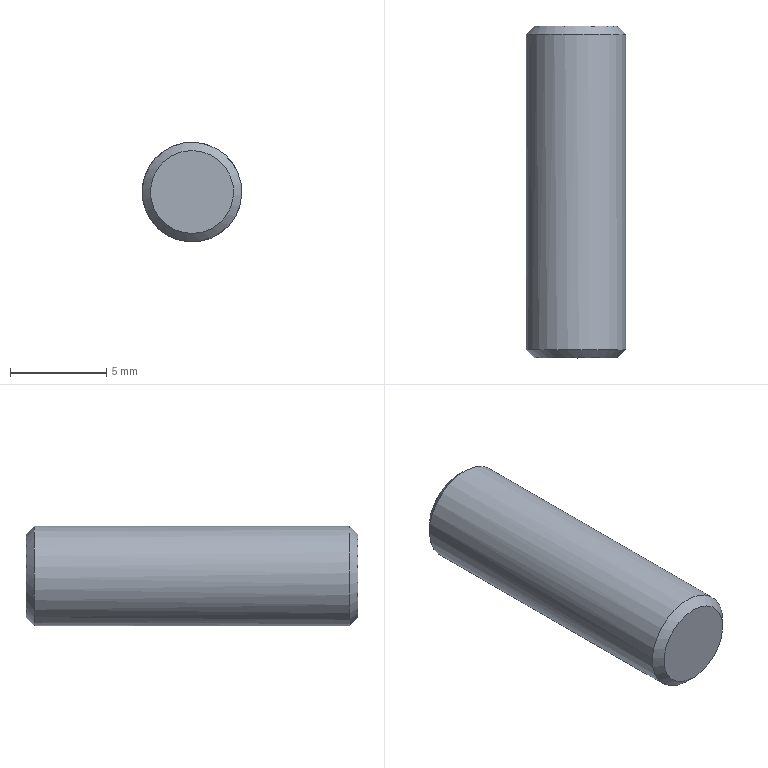Component | NX | 6_LOCATING_PIN | 1 solid | 5 faces | box 5.16 x 17.2 x 5.16 mm | volume 357 mm3 | plane 2 | cone 2 | cylinder 1 | commonest cylinder face diameters 5.16 x1
STEP:
#1=CARTESIAN_POINT('',(0.,0.,0.));
#2=DIRECTION('',(0.,0.,1.));
#3=DIRECTION('',(1.,0.,0.));
#4=AXIS2_PLACEMENT_3D('',#1,#2,#3);
#5=CARTESIAN_POINT('',(-93.38,-477.073,-34.452));
#6=VERTEX_POINT('',#5);
#7=CARTESIAN_POINT('',(-95.366,-477.073,-35.275));
#8=DIRECTION('',(0.,1.,0.));
#9=DIRECTION('',(0.9237,0.,0.383));
#10=AXIS2_PLACEMENT_3D('',#7,#8,#9);
#11=CIRCLE('',#10,2.15);
#12=CARTESIAN_POINT('',(-95.366,-477.073,-35.275));
#13=DIRECTION('',(0.,1.,0.));
#14=DIRECTION('',(0.9237,0.,0.383));
#15=AXIS2_PLACEMENT_3D('',#12,#13,#14);
#16=PLANE('',#15);
#17=CARTESIAN_POINT('',(0.,0.));
#18=DIRECTION('',(1.,-0.));
#19=AXIS2_PLACEMENT_2D('',#17,#18);
#20=CIRCLE('',#19,2.15);
#21=(GEOMETRIC_REPRESENTATION_CONTEXT(2)PARAMETRIC_REPRESENTATION_CONTEXT()REPRESENTATION_CONTEXT('',''));
#22=DEFINITIONAL_REPRESENTATION('',(#20),#21);
#23=PCURVE('',#16,#22);
#24=CARTESIAN_POINT('',(-95.366,-477.503,-35.275));
#25=DIRECTION('',(0.,-1.,0.));
#26=DIRECTION('',(-0.9237,0.,-0.383));
#27=AXIS2_PLACEMENT_3D('',#24,#25,#26);
#28=CONICAL_SURFACE('',#27,2.58,0.7854);
#29=CARTESIAN_POINT('',(9.425,-0.43));
#30=DIRECTION('',(-1.,0.));
#31=VECTOR('',#30,1.);
#32=LINE('',#29,#31);
#33=(GEOMETRIC_REPRESENTATION_CONTEXT(2)PARAMETRIC_REPRESENTATION_CONTEXT()REPRESENTATION_CONTEXT('',''));
#34=DEFINITIONAL_REPRESENTATION('',(#32),#33);
#35=PCURVE('',#28,#34);
#36=SURFACE_CURVE('',#11,(#23,#35),.PCURVE_S1.);
#37=EDGE_CURVE('',#6,#6,#36,.T.);
#38=ORIENTED_EDGE('',*,*,#37,.T.);
#39=EDGE_LOOP('',(#38));
#40=FACE_BOUND('',#39,.T.);
#41=ADVANCED_FACE('',(#40),#16,.T.);
#42=CARTESIAN_POINT('',(-97.352,-494.273,-36.099));
#43=VERTEX_POINT('',#42);
#44=CARTESIAN_POINT('',(-95.366,-494.273,-35.275));
#45=DIRECTION('',(0.,-1.,0.));
#46=DIRECTION('',(-0.9237,0.,-0.383));
#47=AXIS2_PLACEMENT_3D('',#44,#45,#46);
#48=CIRCLE('',#47,2.15);
#49=CARTESIAN_POINT('',(-95.366,-494.273,-35.275));
#50=DIRECTION('',(0.,-1.,0.));
#51=DIRECTION('',(-0.9237,0.,-0.383));
#52=AXIS2_PLACEMENT_3D('',#49,#50,#51);
#53=PLANE('',#52);
#54=CARTESIAN_POINT('',(0.,0.));
#55=DIRECTION('',(1.,0.));
#56=AXIS2_PLACEMENT_2D('',#54,#55);
#57=CIRCLE('',#56,2.15);
#58=(GEOMETRIC_REPRESENTATION_CONTEXT(2)PARAMETRIC_REPRESENTATION_CONTEXT()REPRESENTATION_CONTEXT('',''));
#59=DEFINITIONAL_REPRESENTATION('',(#57),#58);
#60=PCURVE('',#53,#59);
#61=CARTESIAN_POINT('',(-95.366,-493.843,-35.275));
#62=DIRECTION('',(0.,1.,0.));
#63=DIRECTION('',(0.9237,0.,0.383));
#64=AXIS2_PLACEMENT_3D('',#61,#62,#63);
#65=CONICAL_SURFACE('',#64,2.58,0.7854);
#66=CARTESIAN_POINT('',(9.425,-0.43));
#67=DIRECTION('',(-1.,0.));
#68=VECTOR('',#67,1.);
#69=LINE('',#66,#68);
#70=(GEOMETRIC_REPRESENTATION_CONTEXT(2)PARAMETRIC_REPRESENTATION_CONTEXT()REPRESENTATION_CONTEXT('',''));
#71=DEFINITIONAL_REPRESENTATION('',(#69),#70);
#72=PCURVE('',#65,#71);
#73=SURFACE_CURVE('',#48,(#60,#72),.PCURVE_S1.);
#74=EDGE_CURVE('',#43,#43,#73,.T.);
#75=ORIENTED_EDGE('',*,*,#74,.T.);
#76=EDGE_LOOP('',(#75));
#77=FACE_BOUND('',#76,.T.);
#78=ADVANCED_FACE('',(#77),#53,.T.);
#79=CARTESIAN_POINT('',(-97.749,-493.843,-36.264));
#80=VERTEX_POINT('',#79);
#81=CARTESIAN_POINT('',(-92.982,-493.843,-34.287));
#82=VERTEX_POINT('',#81);
#83=CARTESIAN_POINT('',(-95.366,-493.843,-35.275));
#84=DIRECTION('',(0.,1.,0.));
#85=DIRECTION('',(-0.9237,0.,-0.383));
#86=AXIS2_PLACEMENT_3D('',#83,#84,#85);
#87=CIRCLE('',#86,2.58);
#88=CARTESIAN_POINT('',(-95.366,-494.273,-35.275));
#89=DIRECTION('',(0.,1.,0.));
#90=DIRECTION('',(0.9237,0.,0.383));
#91=AXIS2_PLACEMENT_3D('',#88,#89,#90);
#92=CYLINDRICAL_SURFACE('',#91,2.58);
#93=CARTESIAN_POINT('',(3.142,0.43));
#94=DIRECTION('',(1.,0.));
#95=VECTOR('',#94,1.);
#96=LINE('',#93,#95);
#97=(GEOMETRIC_REPRESENTATION_CONTEXT(2)PARAMETRIC_REPRESENTATION_CONTEXT()REPRESENTATION_CONTEXT('',''));
#98=DEFINITIONAL_REPRESENTATION('',(#96),#97);
#99=PCURVE('',#92,#98);
#100=CARTESIAN_POINT('',(3.142,0.));
#101=DIRECTION('',(1.,0.));
#102=VECTOR('',#101,1.);
#103=LINE('',#100,#102);
#104=(GEOMETRIC_REPRESENTATION_CONTEXT(2)PARAMETRIC_REPRESENTATION_CONTEXT()REPRESENTATION_CONTEXT('',''));
#105=DEFINITIONAL_REPRESENTATION('',(#103),#104);
#106=PCURVE('',#65,#105);
#107=SURFACE_CURVE('',#87,(#99,#106),.PCURVE_S1.);
#108=EDGE_CURVE('',#80,#82,#107,.T.);
#109=ORIENTED_EDGE('',*,*,#108,.T.);
#110=CARTESIAN_POINT('',(-92.982,-477.503,-34.287));
#111=VERTEX_POINT('',#110);
#112=CARTESIAN_POINT('',(-92.982,-493.843,-34.287));
#113=CARTESIAN_POINT('',(-92.982,-477.503,-34.287));
#114=B_SPLINE_CURVE_WITH_KNOTS('',1,(#112,#113),.UNSPECIFIED.,.F.,.F.,(2,2),(0.43,16.77),.PIECEWISE_BEZIER_KNOTS.);
#115=CARTESIAN_POINT('',(6.283,0.));
#116=DIRECTION('',(0.,1.));
#117=VECTOR('',#116,1.);
#118=LINE('',#115,#117);
#119=(GEOMETRIC_REPRESENTATION_CONTEXT(2)PARAMETRIC_REPRESENTATION_CONTEXT()REPRESENTATION_CONTEXT('',''));
#120=DEFINITIONAL_REPRESENTATION('',(#118),#119);
#121=PCURVE('',#92,#120);
#122=CARTESIAN_POINT('',(0.,0.));
#123=DIRECTION('',(0.,1.));
#124=VECTOR('',#123,1.);
#125=LINE('',#122,#124);
#126=(GEOMETRIC_REPRESENTATION_CONTEXT(2)PARAMETRIC_REPRESENTATION_CONTEXT()REPRESENTATION_CONTEXT('',''));
#127=DEFINITIONAL_REPRESENTATION('',(#125),#126);
#128=PCURVE('',#92,#127);
#129=SEAM_CURVE('',#114,(#121,#128),.PCURVE_S1.);
#130=EDGE_CURVE('',#82,#111,#129,.T.);
#131=ORIENTED_EDGE('',*,*,#130,.T.);
#132=CARTESIAN_POINT('',(-95.366,-477.503,-35.275));
#133=DIRECTION('',(0.,-1.,0.));
#134=DIRECTION('',(0.9237,0.,0.383));
#135=AXIS2_PLACEMENT_3D('',#132,#133,#134);
#136=CIRCLE('',#135,2.58);
#137=CARTESIAN_POINT('',(6.283,16.77));
#138=DIRECTION('',(-1.,0.));
#139=VECTOR('',#138,1.);
#140=LINE('',#137,#139);
#141=(GEOMETRIC_REPRESENTATION_CONTEXT(2)PARAMETRIC_REPRESENTATION_CONTEXT()REPRESENTATION_CONTEXT('',''));
#142=DEFINITIONAL_REPRESENTATION('',(#140),#141);
#143=PCURVE('',#92,#142);
#144=CARTESIAN_POINT('',(3.142,-0.));
#145=DIRECTION('',(1.,0.));
#146=VECTOR('',#145,1.);
#147=LINE('',#144,#146);
#148=(GEOMETRIC_REPRESENTATION_CONTEXT(2)PARAMETRIC_REPRESENTATION_CONTEXT()REPRESENTATION_CONTEXT('',''));
#149=DEFINITIONAL_REPRESENTATION('',(#147),#148);
#150=PCURVE('',#28,#149);
#151=SURFACE_CURVE('',#136,(#143,#150),.PCURVE_S1.);
#152=EDGE_CURVE('',#111,#111,#151,.T.);
#153=ORIENTED_EDGE('',*,*,#152,.T.);
#154=ORIENTED_EDGE('',*,*,#130,.F.);
#155=CARTESIAN_POINT('',(-95.366,-493.843,-35.275));
#156=DIRECTION('',(0.,1.,0.));
#157=DIRECTION('',(-0.9237,0.,-0.383));
#158=AXIS2_PLACEMENT_3D('',#155,#156,#157);
#159=CIRCLE('',#158,2.58);
#160=CARTESIAN_POINT('',(-3.142,0.43));
#161=DIRECTION('',(1.,0.));
#162=VECTOR('',#161,1.);
#163=LINE('',#160,#162);
#164=(GEOMETRIC_REPRESENTATION_CONTEXT(2)PARAMETRIC_REPRESENTATION_CONTEXT()REPRESENTATION_CONTEXT('',''));
#165=DEFINITIONAL_REPRESENTATION('',(#163),#164);
#166=PCURVE('',#92,#165);
#167=CARTESIAN_POINT('',(3.142,0.));
#168=DIRECTION('',(1.,0.));
#169=VECTOR('',#168,1.);
#170=LINE('',#167,#169);
#171=(GEOMETRIC_REPRESENTATION_CONTEXT(2)PARAMETRIC_REPRESENTATION_CONTEXT()REPRESENTATION_CONTEXT('',''));
#172=DEFINITIONAL_REPRESENTATION('',(#170),#171);
#173=PCURVE('',#65,#172);
#174=SURFACE_CURVE('',#159,(#166,#173),.PCURVE_S1.);
#175=EDGE_CURVE('',#82,#80,#174,.T.);
#176=ORIENTED_EDGE('',*,*,#175,.T.);
#177=EDGE_LOOP('',(#109,#131,#153,#154,#176));
#178=FACE_BOUND('',#177,.T.);
#179=ADVANCED_FACE('',(#178),#92,.T.);
#180=ORIENTED_EDGE('',*,*,#74,.F.);
#181=CARTESIAN_POINT('',(-97.352,-494.273,-36.099));
#182=CARTESIAN_POINT('',(-97.749,-493.843,-36.264));
#183=B_SPLINE_CURVE_WITH_KNOTS('',1,(#181,#182),.UNSPECIFIED.,.F.,.F.,(2,2),(-0.6081,0.),.PIECEWISE_BEZIER_KNOTS.);
#184=CARTESIAN_POINT('',(9.425,0.));
#185=DIRECTION('',(0.,1.));
#186=VECTOR('',#185,1.);
#187=LINE('',#184,#186);
#188=(GEOMETRIC_REPRESENTATION_CONTEXT(2)PARAMETRIC_REPRESENTATION_CONTEXT()REPRESENTATION_CONTEXT('',''));
#189=DEFINITIONAL_REPRESENTATION('',(#187),#188);
#190=PCURVE('',#65,#189);
#191=CARTESIAN_POINT('',(3.142,0.));
#192=DIRECTION('',(0.,1.));
#193=VECTOR('',#192,1.);
#194=LINE('',#191,#193);
#195=(GEOMETRIC_REPRESENTATION_CONTEXT(2)PARAMETRIC_REPRESENTATION_CONTEXT()REPRESENTATION_CONTEXT('',''));
#196=DEFINITIONAL_REPRESENTATION('',(#194),#195);
#197=PCURVE('',#65,#196);
#198=SEAM_CURVE('',#183,(#190,#197),.PCURVE_S1.);
#199=EDGE_CURVE('',#43,#80,#198,.T.);
#200=ORIENTED_EDGE('',*,*,#199,.T.);
#201=ORIENTED_EDGE('',*,*,#175,.F.);
#202=ORIENTED_EDGE('',*,*,#108,.F.);
#203=ORIENTED_EDGE('',*,*,#199,.F.);
#204=EDGE_LOOP('',(#180,#200,#201,#202,#203));
#205=FACE_BOUND('',#204,.T.);
#206=ADVANCED_FACE('',(#205),#65,.T.);
#207=ORIENTED_EDGE('',*,*,#37,.F.);
#208=CARTESIAN_POINT('',(-93.38,-477.073,-34.452));
#209=CARTESIAN_POINT('',(-92.982,-477.503,-34.287));
#210=B_SPLINE_CURVE_WITH_KNOTS('',1,(#208,#209),.UNSPECIFIED.,.F.,.F.,(2,2),(-0.6081,-0.),.PIECEWISE_BEZIER_KNOTS.);
#211=CARTESIAN_POINT('',(9.425,0.));
#212=DIRECTION('',(0.,1.));
#213=VECTOR('',#212,1.);
#214=LINE('',#211,#213);
#215=(GEOMETRIC_REPRESENTATION_CONTEXT(2)PARAMETRIC_REPRESENTATION_CONTEXT()REPRESENTATION_CONTEXT('',''));
#216=DEFINITIONAL_REPRESENTATION('',(#214),#215);
#217=PCURVE('',#28,#216);
#218=CARTESIAN_POINT('',(3.142,0.));
#219=DIRECTION('',(0.,1.));
#220=VECTOR('',#219,1.);
#221=LINE('',#218,#220);
#222=(GEOMETRIC_REPRESENTATION_CONTEXT(2)PARAMETRIC_REPRESENTATION_CONTEXT()REPRESENTATION_CONTEXT('',''));
#223=DEFINITIONAL_REPRESENTATION('',(#221),#222);
#224=PCURVE('',#28,#223);
#225=SEAM_CURVE('',#210,(#217,#224),.PCURVE_S1.);
#226=EDGE_CURVE('',#6,#111,#225,.T.);
#227=ORIENTED_EDGE('',*,*,#226,.T.);
#228=ORIENTED_EDGE('',*,*,#152,.F.);
#229=ORIENTED_EDGE('',*,*,#226,.F.);
#230=EDGE_LOOP('',(#207,#227,#228,#229));
#231=FACE_BOUND('',#230,.T.);
#232=ADVANCED_FACE('',(#231),#28,.T.);
#233=CLOSED_SHELL('',(#41,#78,#179,#206,#232));
#234=MANIFOLD_SOLID_BREP('',#233);
#235=(LENGTH_UNIT()NAMED_UNIT(*)SI_UNIT(.MILLI.,.METRE.));
#236=UNCERTAINTY_MEASURE_WITH_UNIT(LENGTH_MEASURE(0.00001),#235,'','');
#237=(NAMED_UNIT(*)PLANE_ANGLE_UNIT()SI_UNIT($,.RADIAN.));
#238=(NAMED_UNIT(*)SI_UNIT($,.STERADIAN.)SOLID_ANGLE_UNIT());
#239=(GEOMETRIC_REPRESENTATION_CONTEXT(3)GLOBAL_UNCERTAINTY_ASSIGNED_CONTEXT((#236))GLOBAL_UNIT_ASSIGNED_CONTEXT((#235,#237,#238))REPRESENTATION_CONTEXT('',''));
#240=ADVANCED_BREP_SHAPE_REPRESENTATION('',(#4,#234),#239);